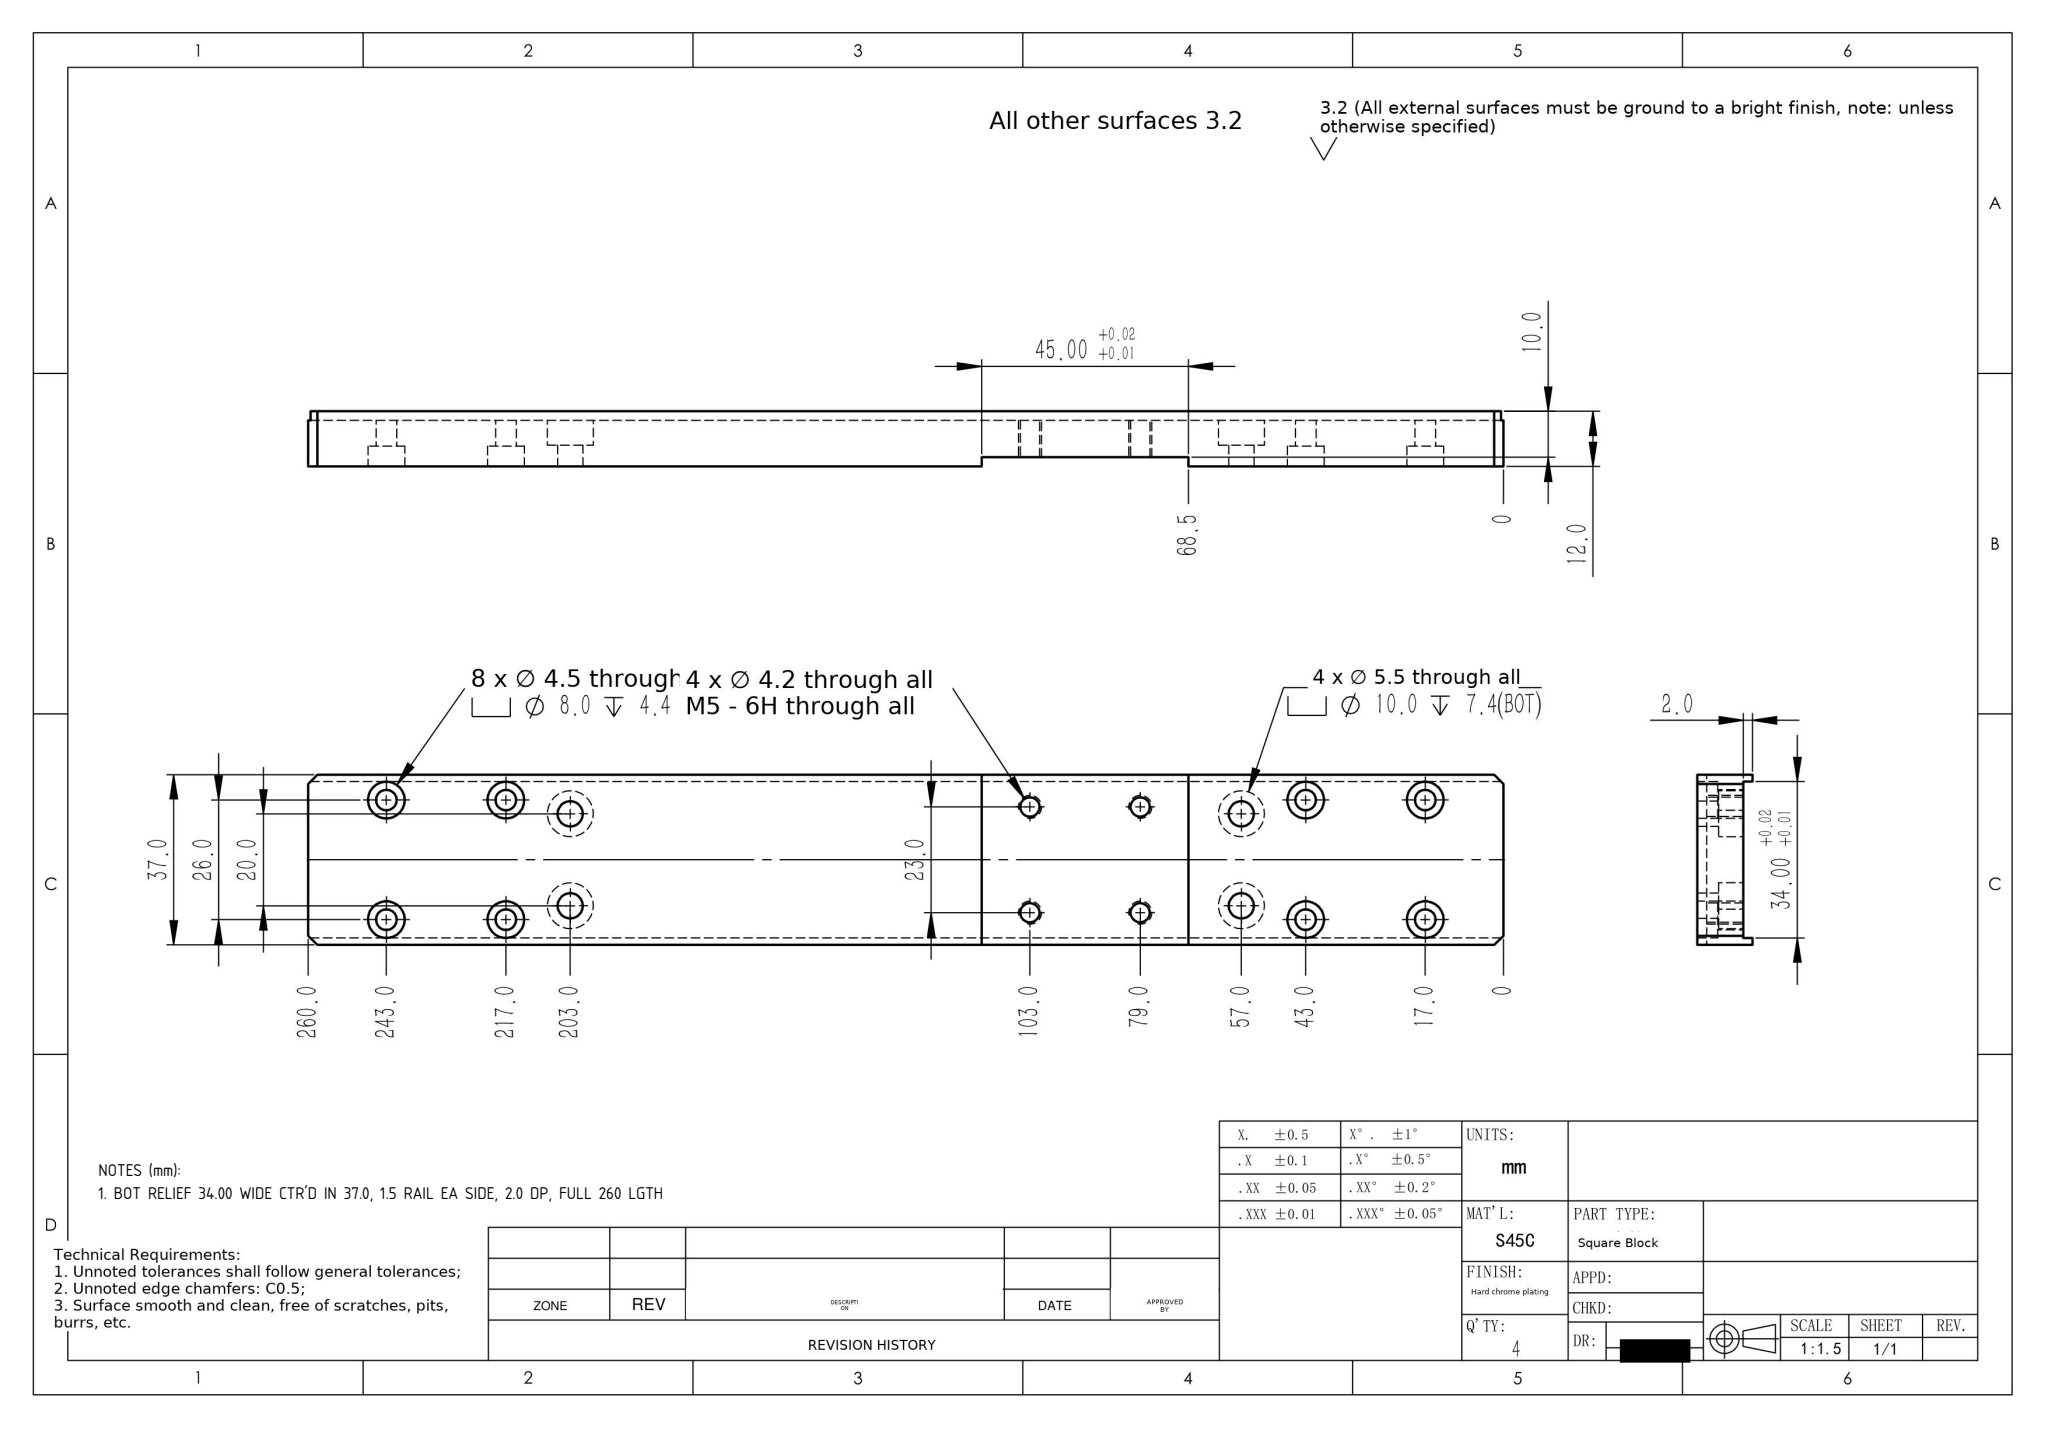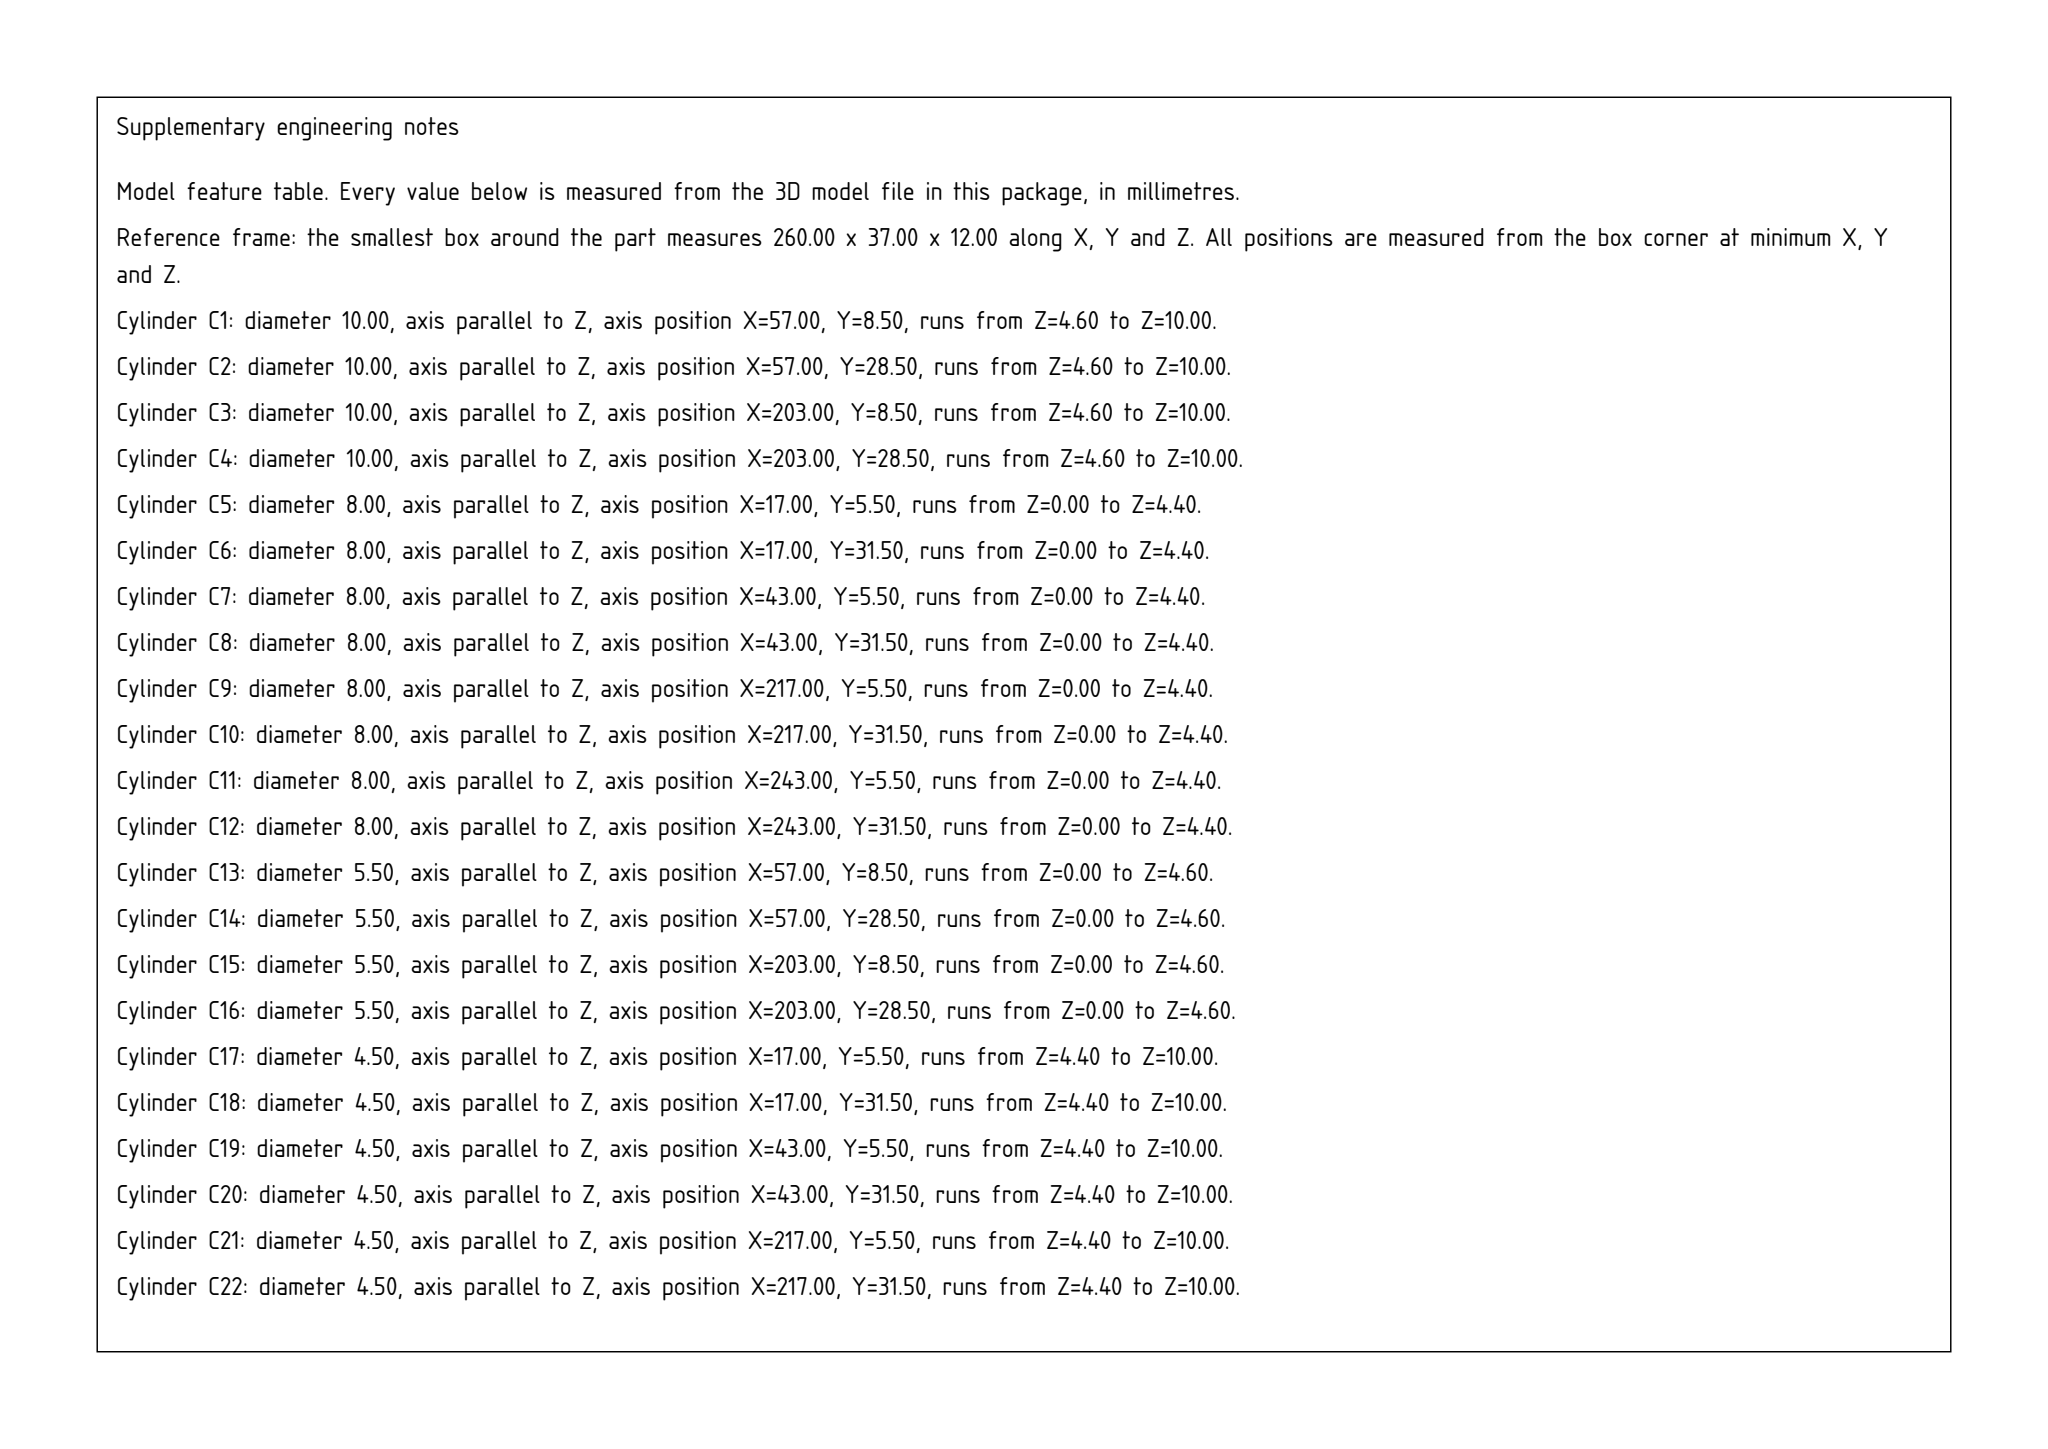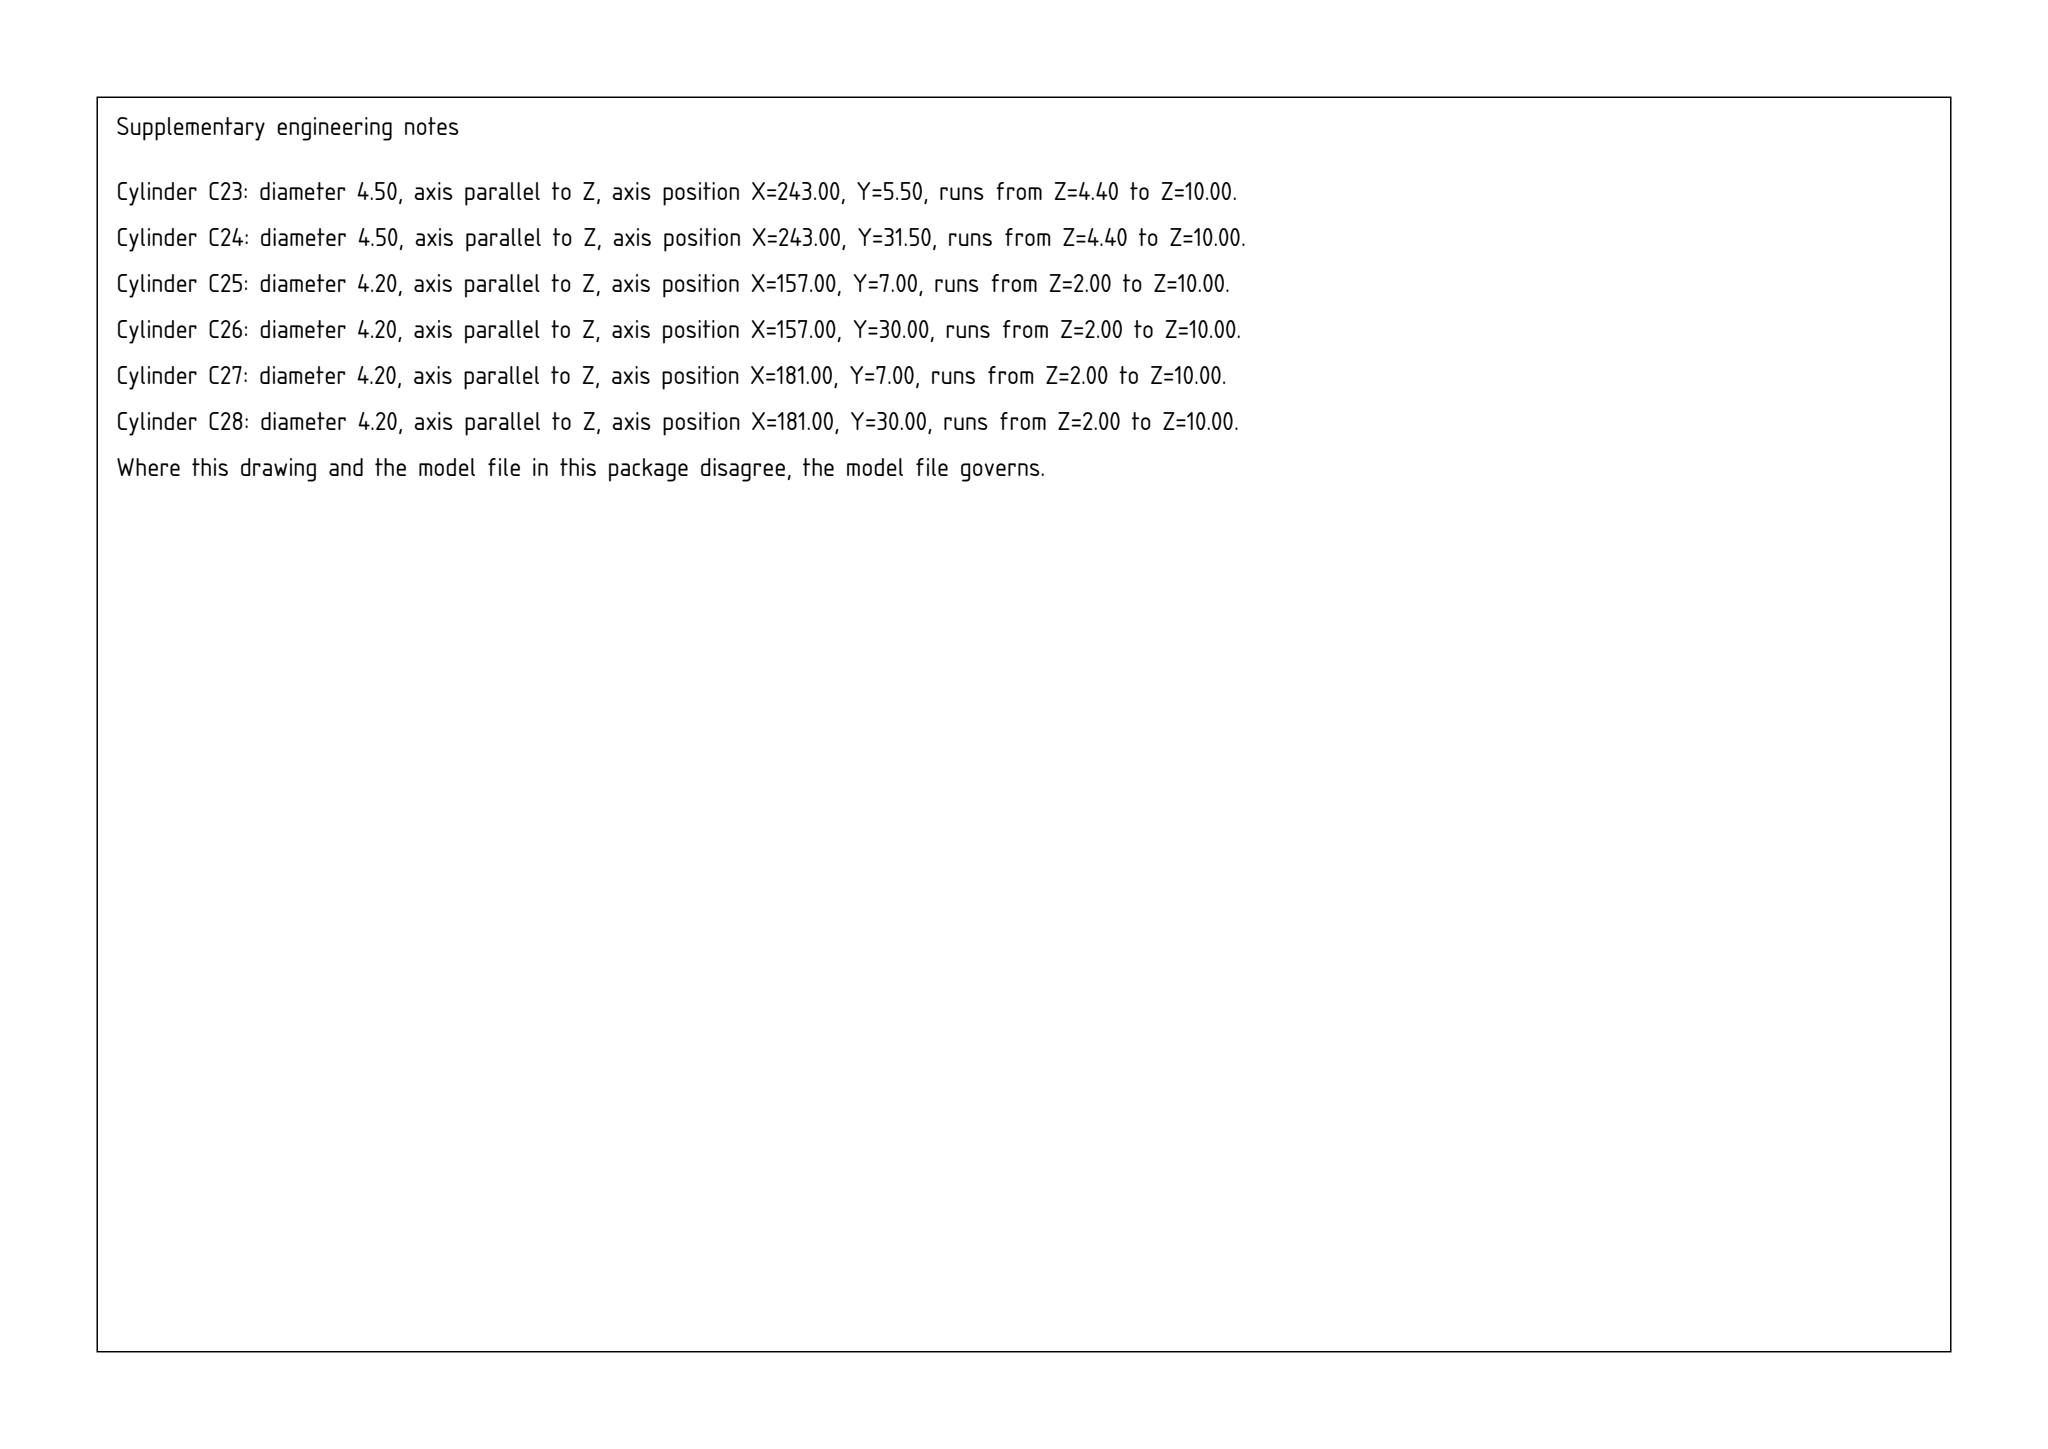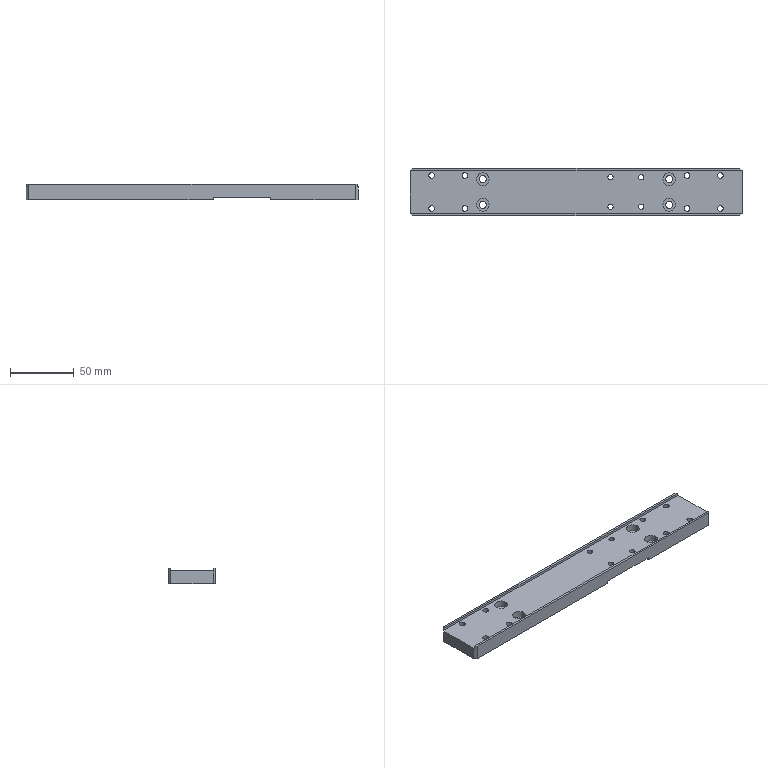Part | SolidWorks | mm | 1 solid | 86 faces | box 260 x 37 x 12 mm | volume 89276 mm3 | cylinder 56 | plane 30 | commonest cylinder face diameters 8 x16 4.5 x16 10 x8 5.5 x8 4.2 x8
Drawing notes:
BOT RELIEF 34.00 WIDE CTR'D IN 37.0, 1.5 RAIL EA SIDE, 2.0 DP, FULL 260 LGTH | from the solid: y-planes 0/1.5/35.5/37.0 give 34.00 ctr'd in 37.0; z-plane 2.0 above bottom; x 0 to 260.0
build123d program:
from build123d import *

# Parameters (mm, degrees)
SKETCH1_W                                       = 260
SKETCH1_H                                       = 37
BOSS_EXTRUDE1_DEPTH                             = 12
M5_TAPPED_HOLE1_D                               = 4.2
M5_HEX_SOCKET_HEAD_CAP_SCREW_CBORE1_D           = 5.5
M5_HEX_SOCKET_HEAD_CAP_SCREW_CBORE1_CBORE_D     = 10
M5_HEX_SOCKET_HEAD_CAP_SCREW_CBORE1_CBORE_DEPTH = 7.4
M4_HEX_SOCKET_HEAD_CAP_SCREW_CBORE1_D           = 4.5
M4_HEX_SOCKET_HEAD_CAP_SCREW_CBORE1_CBORE_D     = 8
M4_HEX_SOCKET_HEAD_CAP_SCREW_CBORE1_CBORE_DEPTH = 4.4
SKETCH10_W                                      = 260
SKETCH10_H                                      = 34
CUT_EXTRUDE1_DEPTH                              = 2
SKETCH11_W                                      = 45
SKETCH11_H                                      = 37
CUT_EXTRUDE2_DEPTH                              = 2
CHAMFER1_SIZE                                   = 2


with BuildPart() as part:
    # Sketch1 → Boss-Extrude1 (new body)
    with BuildSketch(Plane.XY):
        Rectangle(SKETCH1_W, SKETCH1_H)
    extrude(amount=BOSS_EXTRUDE1_DEPTH)

    # M5 Tapped Hole1 (through all)
    with Locations(Plane(origin=(0, 0, 0), x_dir=(-1, 0, 0), z_dir=(0, 0, -1))):
        with Locations((-51, -11.5), (-51, 11.5), (-27, 11.5), (-27, -11.5)):
            Hole(M5_TAPPED_HOLE1_D / 2)

    # M5 Hex Socket Head Cap Screw CBORE1 (through all)
    with Locations(Plane.XY.offset(12)):
        with Locations((-73, 10), (-73, -10), (73, 10), (73, -10)):
            CounterBoreHole(M5_HEX_SOCKET_HEAD_CAP_SCREW_CBORE1_D / 2, M5_HEX_SOCKET_HEAD_CAP_SCREW_CBORE1_CBORE_D / 2, M5_HEX_SOCKET_HEAD_CAP_SCREW_CBORE1_CBORE_DEPTH)

    # M4 Hex Socket Head Cap Screw CBORE1 (through all)
    with Locations(Plane(origin=(0, 0, 0), x_dir=(-1, 0, 0), z_dir=(0, 0, -1))):
        with Locations((87, -13), (87, 13), (113, 13), (113, -13), (-113, -13), (-87, -13), (-113, 13), (-87, 13)):
            CounterBoreHole(M4_HEX_SOCKET_HEAD_CAP_SCREW_CBORE1_D / 2, M4_HEX_SOCKET_HEAD_CAP_SCREW_CBORE1_CBORE_D / 2, M4_HEX_SOCKET_HEAD_CAP_SCREW_CBORE1_CBORE_DEPTH)

    # Sketch10 → Cut-Extrude1 (cut)
    with BuildSketch(Plane.XY.offset(12)):
        Rectangle(SKETCH10_W, SKETCH10_H)
    extrude(amount=-CUT_EXTRUDE1_DEPTH, mode=Mode.SUBTRACT)

    # Sketch11 → Cut-Extrude2 (cut)
    with BuildSketch(Plane(origin=(0, 0, 0), x_dir=(-1, 0, 0), z_dir=(0, 0, -1))):
        with Locations((-39, 0)):
            Rectangle(SKETCH11_W, SKETCH11_H)
    extrude(amount=-CUT_EXTRUDE2_DEPTH, mode=Mode.SUBTRACT)

    # Chamfer1
    chamfer1_edges = [part.edges().sort_by_distance(p)[0] for p in [
        (-130, -18.5, 6),
        (-130, 18.5, 6),
        (130, -18.5, 6),
        (130, 18.5, 6),
    ]]
    chamfer(chamfer1_edges, length=CHAMFER1_SIZE)


solid = part.part